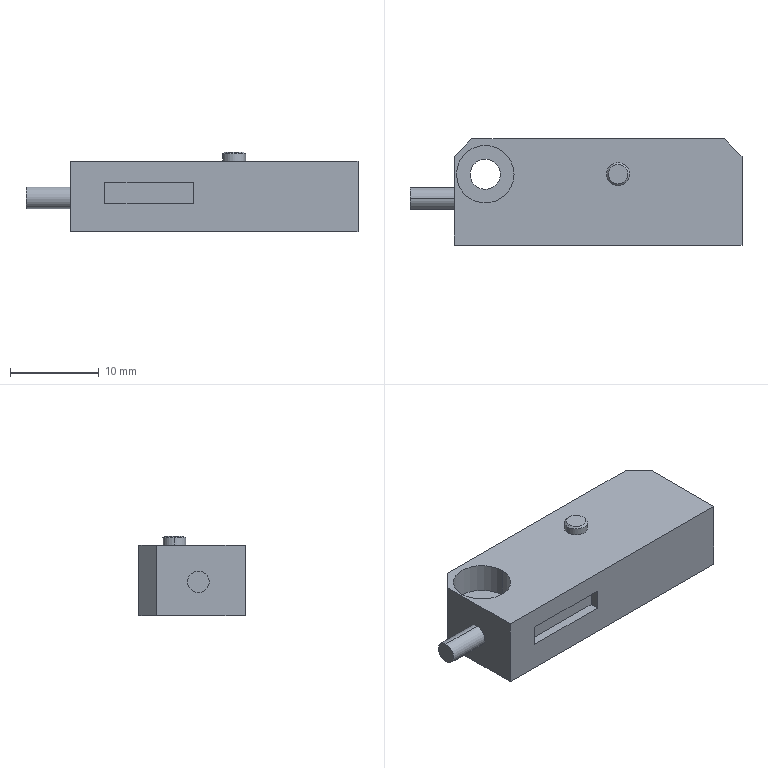Component | SolidWorks | FPJ-D21-1 | 1 solid | 26 faces | box 37.5 x 12 x 9 mm | volume 2938 mm3 | plane 16 | cylinder 8 | cone 2 | commonest cylinder face diameters 6.5 x2 3.4 x2 2.442 x2 2.6 x2
build123d program:
from build123d import *

# Parameters (mm, degrees)
SKETCH1_W                                       = 32.5
SKETCH1_H                                       = 12
BOSS_EXTRUDE1_DEPTH                             = 8
SKETCH2_R                                       = 1.3
BOSS_EXTRUDE2_DEPTH                             = 1
CHAMFER1_SIZE                                   = 2
SKETCH3_R                                       = 1.221
BOSS_EXTRUDE3_DEPTH                             = 5
M3_HEX_SOCKET_HEAD_CAP_SCREW_CBORE1_D           = 3.4
M3_HEX_SOCKET_HEAD_CAP_SCREW_CBORE1_CBORE_D     = 6.5
M3_HEX_SOCKET_HEAD_CAP_SCREW_CBORE1_CBORE_DEPTH = 3.4
BOSS_EXTRUDE4_START                             = 1
SKETCH6_R                                       = 1.3
BOSS_EXTRUDE4_DEPTH                             = 1
CHAMFER2_SIZE                                   = 0.2
SKETCH7_W                                       = 9.996
SKETCH7_H                                       = 2.373
CUT_EXTRUDE1_DEPTH                              = 1
PINSTUBRELIEF_SKETCH_R                          = 2
PINSTUBRELIEF_DEPTH                             = 2


with BuildPart() as part:
    # Sketch1 → Boss-Extrude1 (new body)
    with BuildSketch(Plane.XY):
        with Locations((-16.25, 6)):
            Rectangle(SKETCH1_W, SKETCH1_H)
    extrude(amount=BOSS_EXTRUDE1_DEPTH)

    # Sketch2 → Boss-Extrude2 (add)
    with BuildSketch(Plane.XY.offset(8)):
        with Locations((-14, 8)):
            Circle(SKETCH2_R)
    extrude(amount=BOSS_EXTRUDE2_DEPTH)

    # Chamfer1
    chamfer1_edges = [part.edges().sort_by_distance(p)[0] for p in [
        (-32.5, 12, 4),
        (0, 12, 4),
    ]]
    chamfer(chamfer1_edges, length=CHAMFER1_SIZE)

    # Sketch3 → Boss-Extrude3 (add)
    with BuildSketch(Plane.ZY.offset(32.5)):
        with Locations(Location((3.84, 5.275, 0), (0, 0, 180))):
            Circle(SKETCH3_R)
    extrude(amount=BOSS_EXTRUDE3_DEPTH)

    # M3 Hex Socket Head Cap Screw CBORE1 (through all)
    with Locations(Plane.XY.offset(8)):
        with Locations((-29, 8)):
            CounterBoreHole(M3_HEX_SOCKET_HEAD_CAP_SCREW_CBORE1_D / 2, M3_HEX_SOCKET_HEAD_CAP_SCREW_CBORE1_CBORE_D / 2, M3_HEX_SOCKET_HEAD_CAP_SCREW_CBORE1_CBORE_DEPTH)

    # Sketch6 → Boss-Extrude4 (add)
    with BuildSketch(Plane(origin=(0, 0, 0), x_dir=(-1, 0, 0), z_dir=(0, 0, -1)).offset(BOSS_EXTRUDE4_START)):
        with Locations(Location((14, 8, 0), (0, 0, 180))):
            Circle(SKETCH6_R)
    extrude(amount=-BOSS_EXTRUDE4_DEPTH)

    # Chamfer2
    chamfer2_edges = [part.edges().sort_by_distance(p)[0] for p in [
        (-15.3, 8, 9),
        (-15.3, 8, -1),
    ]]
    chamfer(chamfer2_edges, length=CHAMFER2_SIZE)

    # Sketch7 → Cut-Extrude1 (cut)
    with BuildSketch(Plane.XZ):
        with Locations((-23.593, 4.408)):
            Rectangle(SKETCH7_W, SKETCH7_H)
    extrude(amount=-CUT_EXTRUDE1_DEPTH, mode=Mode.SUBTRACT)

    # PinStubRelief_Sketch → PinStubRelief (cut)
    with BuildSketch(Plane.XY):
        with Locations((-14, 8)):
            Circle(PINSTUBRELIEF_SKETCH_R)
    extrude(amount=-PINSTUBRELIEF_DEPTH, mode=Mode.SUBTRACT)


solid = part.part

# Placed as in the assembly
solid = solid.moved(Location((215.5, -74, 1001.634), (0, 0, 0)))
STEP:
#1=COLOUR_RGB('',0.7922,0.8196,0.9333);
#2=FILL_AREA_STYLE_COLOUR('',#1);
#3=FILL_AREA_STYLE('',(#2));
#4=SURFACE_STYLE_FILL_AREA(#3);
#5=SURFACE_SIDE_STYLE('',(#4));
#6=SURFACE_STYLE_USAGE(.BOTH.,#5);
#7=PRESENTATION_STYLE_ASSIGNMENT((#6));
#8=CARTESIAN_POINT('',(7.976,-2.598,39.789));
#9=VERTEX_POINT('',#8);
#10=CARTESIAN_POINT('',(7.89,-2.598,39.789));
#11=VERTEX_POINT('',#10);
#12=CARTESIAN_POINT('',(7.933,-2.598,39.789));
#13=DIRECTION('',(0.,0.,1.));
#14=DIRECTION('',(1.,0.,0.));
#15=AXIS2_PLACEMENT_3D('',#12,#13,#14);
#16=CIRCLE('',#15,0.04331);
#17=EDGE_CURVE('',#9,#11,#16,.T.);
#18=ORIENTED_EDGE('',*,*,#17,.F.);
#19=CARTESIAN_POINT('',(7.984,-2.598,39.781));
#20=VERTEX_POINT('',#19);
#21=CARTESIAN_POINT('',(7.976,-2.598,39.789));
#22=DIRECTION('',(0.7071,0.,-0.7071));
#23=VECTOR('',#22,39.37);
#24=LINE('',#21,#23);
#25=EDGE_CURVE('',#9,#20,#24,.T.);
#26=ORIENTED_EDGE('',*,*,#25,.T.);
#27=CARTESIAN_POINT('',(7.882,-2.598,39.781));
#28=VERTEX_POINT('',#27);
#29=CARTESIAN_POINT('',(7.933,-2.598,39.781));
#30=DIRECTION('',(0.,0.,-1.));
#31=DIRECTION('',(1.,0.,0.));
#32=AXIS2_PLACEMENT_3D('',#29,#30,#31);
#33=CIRCLE('',#32,0.05118);
#34=EDGE_CURVE('',#28,#20,#33,.T.);
#35=ORIENTED_EDGE('',*,*,#34,.F.);
#36=CARTESIAN_POINT('',(7.89,-2.598,39.789));
#37=DIRECTION('',(-0.7071,0.,-0.7071));
#38=VECTOR('',#37,39.37);
#39=LINE('',#36,#38);
#40=EDGE_CURVE('',#11,#28,#39,.T.);
#41=ORIENTED_EDGE('',*,*,#40,.F.);
#42=EDGE_LOOP('',(#18,#26,#35,#41));
#43=FACE_OUTER_BOUND('',#42,.T.);
#44=CARTESIAN_POINT('',(7.933,-2.598,39.789));
#45=DIRECTION('',(0.,0.,-1.));
#46=DIRECTION('',(-1.,0.,0.));
#47=AXIS2_PLACEMENT_3D('',#44,#45,#46);
#48=CONICAL_SURFACE('',#47,0.04331,0.7854);
#49=ADVANCED_FACE('',(#43),#48,.T.);
#50=CARTESIAN_POINT('',(7.215,-2.598,39.616));
#51=VERTEX_POINT('',#50);
#52=CARTESIAN_POINT('',(7.47,-2.598,39.616));
#53=VERTEX_POINT('',#52);
#54=CARTESIAN_POINT('',(7.343,-2.598,39.616));
#55=DIRECTION('',(0.,0.,1.));
#56=DIRECTION('',(1.,0.,0.));
#57=AXIS2_PLACEMENT_3D('',#54,#55,#56);
#58=CIRCLE('',#57,0.128);
#59=EDGE_CURVE('',#51,#53,#58,.T.);
#60=ORIENTED_EDGE('',*,*,#59,.F.);
#61=CARTESIAN_POINT('',(7.215,-2.598,39.749));
#62=VERTEX_POINT('',#61);
#63=CARTESIAN_POINT('',(7.215,-2.598,39.749));
#64=DIRECTION('',(0.,0.,1.));
#65=VECTOR('',#64,39.37);
#66=LINE('',#63,#65);
#67=EDGE_CURVE('',#51,#62,#66,.T.);
#68=ORIENTED_EDGE('',*,*,#67,.T.);
#69=CARTESIAN_POINT('',(7.47,-2.598,39.749));
#70=VERTEX_POINT('',#69);
#71=CARTESIAN_POINT('',(7.343,-2.598,39.749));
#72=DIRECTION('',(0.,0.,1.));
#73=DIRECTION('',(1.,0.,0.));
#74=AXIS2_PLACEMENT_3D('',#71,#72,#73);
#75=CIRCLE('',#74,0.128);
#76=EDGE_CURVE('',#62,#70,#75,.T.);
#77=ORIENTED_EDGE('',*,*,#76,.T.);
#78=CARTESIAN_POINT('',(7.47,-2.598,39.749));
#79=DIRECTION('',(0.,0.,1.));
#80=VECTOR('',#79,39.37);
#81=LINE('',#78,#80);
#82=EDGE_CURVE('',#53,#70,#81,.T.);
#83=ORIENTED_EDGE('',*,*,#82,.F.);
#84=EDGE_LOOP('',(#60,#68,#77,#83));
#85=FACE_OUTER_BOUND('',#84,.T.);
#86=CARTESIAN_POINT('',(7.343,-2.598,39.749));
#87=DIRECTION('',(0.,0.,1.));
#88=DIRECTION('',(1.,0.,0.));
#89=AXIS2_PLACEMENT_3D('',#86,#87,#88);
#90=CYLINDRICAL_SURFACE('',#89,0.128);
#91=ADVANCED_FACE('',(#85),#90,.F.);
#92=CARTESIAN_POINT('',(7.276,-2.598,39.434));
#93=VERTEX_POINT('',#92);
#94=CARTESIAN_POINT('',(7.409,-2.598,39.434));
#95=VERTEX_POINT('',#94);
#96=CARTESIAN_POINT('',(7.343,-2.598,39.434));
#97=DIRECTION('',(0.,0.,1.));
#98=DIRECTION('',(1.,0.,0.));
#99=AXIS2_PLACEMENT_3D('',#96,#97,#98);
#100=CIRCLE('',#99,0.06693);
#101=EDGE_CURVE('',#93,#95,#100,.T.);
#102=ORIENTED_EDGE('',*,*,#101,.F.);
#103=CARTESIAN_POINT('',(7.276,-2.598,39.616));
#104=VERTEX_POINT('',#103);
#105=CARTESIAN_POINT('',(7.276,-2.598,39.749));
#106=DIRECTION('',(0.,0.,1.));
#107=VECTOR('',#106,39.37);
#108=LINE('',#105,#107);
#109=EDGE_CURVE('',#93,#104,#108,.T.);
#110=ORIENTED_EDGE('',*,*,#109,.T.);
#111=CARTESIAN_POINT('',(7.409,-2.598,39.616));
#112=VERTEX_POINT('',#111);
#113=CARTESIAN_POINT('',(7.343,-2.598,39.616));
#114=DIRECTION('',(0.,0.,1.));
#115=DIRECTION('',(1.,0.,0.));
#116=AXIS2_PLACEMENT_3D('',#113,#114,#115);
#117=CIRCLE('',#116,0.06693);
#118=EDGE_CURVE('',#104,#112,#117,.T.);
#119=ORIENTED_EDGE('',*,*,#118,.T.);
#120=CARTESIAN_POINT('',(7.409,-2.598,39.749));
#121=DIRECTION('',(0.,0.,1.));
#122=VECTOR('',#121,39.37);
#123=LINE('',#120,#122);
#124=EDGE_CURVE('',#95,#112,#123,.T.);
#125=ORIENTED_EDGE('',*,*,#124,.F.);
#126=EDGE_LOOP('',(#102,#110,#119,#125));
#127=FACE_OUTER_BOUND('',#126,.T.);
#128=CARTESIAN_POINT('',(7.343,-2.598,39.749));
#129=DIRECTION('',(0.,0.,1.));
#130=DIRECTION('',(1.,0.,0.));
#131=AXIS2_PLACEMENT_3D('',#128,#129,#130);
#132=CYLINDRICAL_SURFACE('',#131,0.06693);
#133=ADVANCED_FACE('',(#127),#132,.F.);
#134=CARTESIAN_POINT('',(7.008,-2.706,39.634));
#135=VERTEX_POINT('',#134);
#136=CARTESIAN_POINT('',(7.008,-2.706,39.538));
#137=VERTEX_POINT('',#136);
#138=CARTESIAN_POINT('',(7.008,-2.706,39.586));
#139=DIRECTION('',(-1.,0.,0.));
#140=DIRECTION('',(0.,0.,1.));
#141=AXIS2_PLACEMENT_3D('',#138,#139,#140);
#142=CIRCLE('',#141,0.04807);
#143=EDGE_CURVE('',#135,#137,#142,.T.);
#144=ORIENTED_EDGE('',*,*,#143,.F.);
#145=CARTESIAN_POINT('',(7.205,-2.706,39.634));
#146=VERTEX_POINT('',#145);
#147=CARTESIAN_POINT('',(7.008,-2.706,39.634));
#148=DIRECTION('',(1.,0.,0.));
#149=VECTOR('',#148,39.37);
#150=LINE('',#147,#149);
#151=EDGE_CURVE('',#135,#146,#150,.T.);
#152=ORIENTED_EDGE('',*,*,#151,.T.);
#153=CARTESIAN_POINT('',(7.205,-2.706,39.538));
#154=VERTEX_POINT('',#153);
#155=CARTESIAN_POINT('',(7.205,-2.706,39.586));
#156=DIRECTION('',(-1.,0.,0.));
#157=DIRECTION('',(0.,0.,-1.));
#158=AXIS2_PLACEMENT_3D('',#155,#156,#157);
#159=CIRCLE('',#158,0.04807);
#160=EDGE_CURVE('',#146,#154,#159,.T.);
#161=ORIENTED_EDGE('',*,*,#160,.T.);
#162=CARTESIAN_POINT('',(7.008,-2.706,39.538));
#163=DIRECTION('',(1.,0.,0.));
#164=VECTOR('',#163,39.37);
#165=LINE('',#162,#164);
#166=EDGE_CURVE('',#137,#154,#165,.T.);
#167=ORIENTED_EDGE('',*,*,#166,.F.);
#168=EDGE_LOOP('',(#144,#152,#161,#167));
#169=FACE_OUTER_BOUND('',#168,.T.);
#170=CARTESIAN_POINT('',(7.008,-2.706,39.586));
#171=DIRECTION('',(1.,0.,0.));
#172=DIRECTION('',(0.,0.,-1.));
#173=AXIS2_PLACEMENT_3D('',#170,#171,#172);
#174=CYLINDRICAL_SURFACE('',#173,0.04807);
#175=ADVANCED_FACE('',(#169),#174,.T.);
#176=ORIENTED_EDGE('',*,*,#34,.T.);
#177=CARTESIAN_POINT('',(7.984,-2.598,39.749));
#178=VERTEX_POINT('',#177);
#179=CARTESIAN_POINT('',(7.984,-2.598,39.789));
#180=DIRECTION('',(0.,0.,-1.));
#181=VECTOR('',#180,39.37);
#182=LINE('',#179,#181);
#183=EDGE_CURVE('',#20,#178,#182,.T.);
#184=ORIENTED_EDGE('',*,*,#183,.T.);
#185=CARTESIAN_POINT('',(7.882,-2.598,39.749));
#186=VERTEX_POINT('',#185);
#187=CARTESIAN_POINT('',(7.933,-2.598,39.749));
#188=DIRECTION('',(0.,0.,1.));
#189=DIRECTION('',(1.,0.,0.));
#190=AXIS2_PLACEMENT_3D('',#187,#188,#189);
#191=CIRCLE('',#190,0.05118);
#192=EDGE_CURVE('',#178,#186,#191,.T.);
#193=ORIENTED_EDGE('',*,*,#192,.T.);
#194=CARTESIAN_POINT('',(7.882,-2.598,39.789));
#195=DIRECTION('',(0.,0.,-1.));
#196=VECTOR('',#195,39.37);
#197=LINE('',#194,#196);
#198=EDGE_CURVE('',#28,#186,#197,.T.);
#199=ORIENTED_EDGE('',*,*,#198,.F.);
#200=EDGE_LOOP('',(#176,#184,#193,#199));
#201=FACE_OUTER_BOUND('',#200,.T.);
#202=CARTESIAN_POINT('',(7.933,-2.598,39.789));
#203=DIRECTION('',(0.,0.,-1.));
#204=DIRECTION('',(-1.,0.,0.));
#205=AXIS2_PLACEMENT_3D('',#202,#203,#204);
#206=CYLINDRICAL_SURFACE('',#205,0.05118);
#207=ADVANCED_FACE('',(#201),#206,.T.);
#208=CARTESIAN_POINT('',(7.343,-2.598,39.434));
#209=DIRECTION('',(0.,0.,1.));
#210=DIRECTION('',(1.,0.,0.));
#211=AXIS2_PLACEMENT_3D('',#208,#209,#210);
#212=CIRCLE('',#211,0.06693);
#213=EDGE_CURVE('',#95,#93,#212,.T.);
#214=ORIENTED_EDGE('',*,*,#213,.T.);
#215=ORIENTED_EDGE('',*,*,#101,.T.);
#216=EDGE_LOOP('',(#214,#215));
#217=FACE_BOUND('',#216,.T.);
#218=CARTESIAN_POINT('',(8.406,-2.441,39.434));
#219=VERTEX_POINT('',#218);
#220=CARTESIAN_POINT('',(7.283,-2.441,39.434));
#221=VERTEX_POINT('',#220);
#222=CARTESIAN_POINT('',(8.484,-2.441,39.434));
#223=DIRECTION('',(-1.,-0.,0.));
#224=VECTOR('',#223,39.37);
#225=LINE('',#222,#224);
#226=EDGE_CURVE('',#219,#221,#225,.T.);
#227=ORIENTED_EDGE('',*,*,#226,.F.);
#228=CARTESIAN_POINT('',(8.484,-2.52,39.434));
#229=VERTEX_POINT('',#228);
#230=CARTESIAN_POINT('',(8.406,-2.441,39.434));
#231=DIRECTION('',(0.7071,-0.7071,0.));
#232=VECTOR('',#231,39.37);
#233=LINE('',#230,#232);
#234=EDGE_CURVE('',#219,#229,#233,.T.);
#235=ORIENTED_EDGE('',*,*,#234,.T.);
#236=CARTESIAN_POINT('',(8.484,-2.913,39.434));
#237=VERTEX_POINT('',#236);
#238=CARTESIAN_POINT('',(8.484,-2.913,39.434));
#239=DIRECTION('',(0.,1.,0.));
#240=VECTOR('',#239,39.37);
#241=LINE('',#238,#240);
#242=EDGE_CURVE('',#237,#229,#241,.T.);
#243=ORIENTED_EDGE('',*,*,#242,.F.);
#244=CARTESIAN_POINT('',(7.205,-2.913,39.434));
#245=VERTEX_POINT('',#244);
#246=CARTESIAN_POINT('',(8.484,-2.913,39.434));
#247=DIRECTION('',(1.,0.,0.));
#248=VECTOR('',#247,39.37);
#249=LINE('',#246,#248);
#250=EDGE_CURVE('',#245,#237,#249,.T.);
#251=ORIENTED_EDGE('',*,*,#250,.F.);
#252=CARTESIAN_POINT('',(7.205,-2.52,39.434));
#253=VERTEX_POINT('',#252);
#254=CARTESIAN_POINT('',(7.205,-2.913,39.434));
#255=DIRECTION('',(0.,-1.,0.));
#256=VECTOR('',#255,39.37);
#257=LINE('',#254,#256);
#258=EDGE_CURVE('',#253,#245,#257,.T.);
#259=ORIENTED_EDGE('',*,*,#258,.F.);
#260=CARTESIAN_POINT('',(7.205,-2.52,39.434));
#261=DIRECTION('',(0.7071,0.7071,0.));
#262=VECTOR('',#261,39.37);
#263=LINE('',#260,#262);
#264=EDGE_CURVE('',#253,#221,#263,.T.);
#265=ORIENTED_EDGE('',*,*,#264,.T.);
#266=EDGE_LOOP('',(#227,#235,#243,#251,#259,#265));
#267=FACE_OUTER_BOUND('',#266,.T.);
#268=CARTESIAN_POINT('',(8.484,-2.913,39.434));
#269=DIRECTION('',(0.,0.,1.));
#270=DIRECTION('',(1.,0.,0.));
#271=AXIS2_PLACEMENT_3D('',#268,#269,#270);
#272=PLANE('',#271);
#273=ADVANCED_FACE('',(#217,#267),#272,.F.);
#274=CARTESIAN_POINT('',(7.205,-2.52,39.749));
#275=VERTEX_POINT('',#274);
#276=CARTESIAN_POINT('',(7.205,-2.913,39.749));
#277=VERTEX_POINT('',#276);
#278=CARTESIAN_POINT('',(7.205,-2.913,39.749));
#279=DIRECTION('',(0.,-1.,0.));
#280=VECTOR('',#279,39.37);
#281=LINE('',#278,#280);
#282=EDGE_CURVE('',#275,#277,#281,.T.);
#283=ORIENTED_EDGE('',*,*,#282,.F.);
#284=CARTESIAN_POINT('',(7.205,-2.52,39.749));
#285=DIRECTION('',(0.,0.,-1.));
#286=VECTOR('',#285,39.37);
#287=LINE('',#284,#286);
#288=EDGE_CURVE('',#275,#253,#287,.T.);
#289=ORIENTED_EDGE('',*,*,#288,.T.);
#290=ORIENTED_EDGE('',*,*,#258,.T.);
#291=CARTESIAN_POINT('',(7.205,-2.913,39.749));
#292=DIRECTION('',(0.,0.,-1.));
#293=VECTOR('',#292,39.37);
#294=LINE('',#291,#293);
#295=EDGE_CURVE('',#277,#245,#294,.T.);
#296=ORIENTED_EDGE('',*,*,#295,.F.);
#297=EDGE_LOOP('',(#283,#289,#290,#296));
#298=FACE_OUTER_BOUND('',#297,.T.);
#299=CARTESIAN_POINT('',(7.205,-2.706,39.586));
#300=DIRECTION('',(-1.,0.,0.));
#301=DIRECTION('',(0.,0.,-1.));
#302=AXIS2_PLACEMENT_3D('',#299,#300,#301);
#303=CIRCLE('',#302,0.04807);
#304=EDGE_CURVE('',#154,#146,#303,.T.);
#305=ORIENTED_EDGE('',*,*,#304,.F.);
#306=ORIENTED_EDGE('',*,*,#160,.F.);
#307=EDGE_LOOP('',(#305,#306));
#308=FACE_BOUND('',#307,.T.);
#309=CARTESIAN_POINT('',(7.205,-2.913,39.749));
#310=DIRECTION('',(1.,0.,0.));
#311=DIRECTION('',(0.,0.,-1.));
#312=AXIS2_PLACEMENT_3D('',#309,#310,#311);
#313=PLANE('',#312);
#314=ADVANCED_FACE('',(#298,#308),#313,.F.);
#315=CARTESIAN_POINT('',(7.343,-2.598,39.749));
#316=DIRECTION('',(0.,0.,1.));
#317=DIRECTION('',(1.,0.,0.));
#318=AXIS2_PLACEMENT_3D('',#315,#316,#317);
#319=CIRCLE('',#318,0.128);
#320=EDGE_CURVE('',#70,#62,#319,.T.);
#321=ORIENTED_EDGE('',*,*,#320,.F.);
#322=ORIENTED_EDGE('',*,*,#76,.F.);
#323=EDGE_LOOP('',(#321,#322));
#324=FACE_BOUND('',#323,.T.);
#325=CARTESIAN_POINT('',(8.484,-2.913,39.749));
#326=VERTEX_POINT('',#325);
#327=CARTESIAN_POINT('',(8.484,-2.52,39.749));
#328=VERTEX_POINT('',#327);
#329=CARTESIAN_POINT('',(8.484,-2.913,39.749));
#330=DIRECTION('',(0.,1.,0.));
#331=VECTOR('',#330,39.37);
#332=LINE('',#329,#331);
#333=EDGE_CURVE('',#326,#328,#332,.T.);
#334=ORIENTED_EDGE('',*,*,#333,.T.);
#335=CARTESIAN_POINT('',(8.406,-2.441,39.749));
#336=VERTEX_POINT('',#335);
#337=CARTESIAN_POINT('',(8.681,-2.717,39.749));
#338=DIRECTION('',(-0.7071,0.7071,0.));
#339=VECTOR('',#338,39.37);
#340=LINE('',#337,#339);
#341=EDGE_CURVE('',#328,#336,#340,.T.);
#342=ORIENTED_EDGE('',*,*,#341,.T.);
#343=CARTESIAN_POINT('',(7.283,-2.441,39.749));
#344=VERTEX_POINT('',#343);
#345=CARTESIAN_POINT('',(8.484,-2.441,39.749));
#346=DIRECTION('',(-1.,-0.,0.));
#347=VECTOR('',#346,39.37);
#348=LINE('',#345,#347);
#349=EDGE_CURVE('',#336,#344,#348,.T.);
#350=ORIENTED_EDGE('',*,*,#349,.T.);
#351=CARTESIAN_POINT('',(7.648,-2.077,39.749));
#352=DIRECTION('',(-0.7071,-0.7071,0.));
#353=VECTOR('',#352,39.37);
#354=LINE('',#351,#353);
#355=EDGE_CURVE('',#344,#275,#354,.T.);
#356=ORIENTED_EDGE('',*,*,#355,.T.);
#357=ORIENTED_EDGE('',*,*,#282,.T.);
#358=CARTESIAN_POINT('',(8.484,-2.913,39.749));
#359=DIRECTION('',(1.,0.,0.));
#360=VECTOR('',#359,39.37);
#361=LINE('',#358,#360);
#362=EDGE_CURVE('',#277,#326,#361,.T.);
#363=ORIENTED_EDGE('',*,*,#362,.T.);
#364=EDGE_LOOP('',(#334,#342,#350,#356,#357,#363));
#365=FACE_OUTER_BOUND('',#364,.T.);
#366=CARTESIAN_POINT('',(7.933,-2.598,39.749));
#367=DIRECTION('',(0.,0.,1.));
#368=DIRECTION('',(1.,0.,0.));
#369=AXIS2_PLACEMENT_3D('',#366,#367,#368);
#370=CIRCLE('',#369,0.05118);
#371=EDGE_CURVE('',#186,#178,#370,.T.);
#372=ORIENTED_EDGE('',*,*,#371,.F.);
#373=ORIENTED_EDGE('',*,*,#192,.F.);
#374=EDGE_LOOP('',(#372,#373));
#375=FACE_BOUND('',#374,.T.);
#376=CARTESIAN_POINT('',(8.484,-2.913,39.749));
#377=DIRECTION('',(0.,0.,1.));
#378=DIRECTION('',(1.,0.,0.));
#379=AXIS2_PLACEMENT_3D('',#376,#377,#378);
#380=PLANE('',#379);
#381=ADVANCED_FACE('',(#324,#365,#375),#380,.T.);
#382=ORIENTED_EDGE('',*,*,#242,.T.);
#383=CARTESIAN_POINT('',(8.484,-2.52,39.749));
#384=DIRECTION('',(0.,0.,1.));
#385=VECTOR('',#384,39.37);
#386=LINE('',#383,#385);
#387=EDGE_CURVE('',#229,#328,#386,.T.);
#388=ORIENTED_EDGE('',*,*,#387,.T.);
#389=ORIENTED_EDGE('',*,*,#333,.F.);
#390=CARTESIAN_POINT('',(8.484,-2.913,39.749));
#391=DIRECTION('',(0.,0.,-1.));
#392=VECTOR('',#391,39.37);
#393=LINE('',#390,#392);
#394=EDGE_CURVE('',#326,#237,#393,.T.);
#395=ORIENTED_EDGE('',*,*,#394,.T.);
#396=EDGE_LOOP('',(#382,#388,#389,#395));
#397=FACE_OUTER_BOUND('',#396,.T.);
#398=CARTESIAN_POINT('',(8.484,-2.913,39.749));
#399=DIRECTION('',(-1.,0.,0.));
#400=DIRECTION('',(0.,0.,1.));
#401=AXIS2_PLACEMENT_3D('',#398,#399,#400);
#402=PLANE('',#401);
#403=ADVANCED_FACE('',(#397),#402,.F.);
#404=ORIENTED_EDGE('',*,*,#349,.F.);
#405=CARTESIAN_POINT('',(8.406,-2.441,39.749));
#406=DIRECTION('',(0.,0.,-1.));
#407=VECTOR('',#406,39.37);
#408=LINE('',#405,#407);
#409=EDGE_CURVE('',#336,#219,#408,.T.);
#410=ORIENTED_EDGE('',*,*,#409,.T.);
#411=ORIENTED_EDGE('',*,*,#226,.T.);
#412=CARTESIAN_POINT('',(7.283,-2.441,39.749));
#413=DIRECTION('',(0.,0.,1.));
#414=VECTOR('',#413,39.37);
#415=LINE('',#412,#414);
#416=EDGE_CURVE('',#221,#344,#415,.T.);
#417=ORIENTED_EDGE('',*,*,#416,.T.);
#418=EDGE_LOOP('',(#404,#410,#411,#417));
#419=FACE_OUTER_BOUND('',#418,.T.);
#420=CARTESIAN_POINT('',(8.484,-2.441,39.749));
#421=DIRECTION('',(0.,-1.,0.));
#422=DIRECTION('',(1.,0.,0.));
#423=AXIS2_PLACEMENT_3D('',#420,#421,#422);
#424=PLANE('',#423);
#425=ADVANCED_FACE('',(#419),#424,.F.);
#426=CARTESIAN_POINT('',(7.359,-2.913,39.561));
#427=VERTEX_POINT('',#426);
#428=CARTESIAN_POINT('',(7.752,-2.913,39.561));
#429=VERTEX_POINT('',#428);
#430=CARTESIAN_POINT('',(7.359,-2.913,39.561));
#431=DIRECTION('',(1.,0.,0.));
#432=VECTOR('',#431,39.37);
#433=LINE('',#430,#432);
#434=EDGE_CURVE('',#427,#429,#433,.T.);
#435=ORIENTED_EDGE('',*,*,#434,.F.);
#436=CARTESIAN_POINT('',(7.359,-2.913,39.655));
#437=VERTEX_POINT('',#436);
#438=CARTESIAN_POINT('',(7.359,-2.913,39.655));
#439=DIRECTION('',(0.,0.,-1.));
#440=VECTOR('',#439,39.37);
#441=LINE('',#438,#440);
#442=EDGE_CURVE('',#437,#427,#441,.T.);
#443=ORIENTED_EDGE('',*,*,#442,.F.);
#444=CARTESIAN_POINT('',(7.752,-2.913,39.655));
#445=VERTEX_POINT('',#444);
#446=CARTESIAN_POINT('',(7.359,-2.913,39.655));
#447=DIRECTION('',(-1.,-0.,0.));
#448=VECTOR('',#447,39.37);
#449=LINE('',#446,#448);
#450=EDGE_CURVE('',#445,#437,#449,.T.);
#451=ORIENTED_EDGE('',*,*,#450,.F.);
#452=CARTESIAN_POINT('',(7.752,-2.913,39.655));
#453=DIRECTION('',(0.,0.,1.));
#454=VECTOR('',#453,39.37);
#455=LINE('',#452,#454);
#456=EDGE_CURVE('',#429,#445,#455,.T.);
#457=ORIENTED_EDGE('',*,*,#456,.F.);
#458=EDGE_LOOP('',(#435,#443,#451,#457));
#459=FACE_BOUND('',#458,.T.);
#460=ORIENTED_EDGE('',*,*,#250,.T.);
#461=ORIENTED_EDGE('',*,*,#394,.F.);
#462=ORIENTED_EDGE('',*,*,#362,.F.);
#463=ORIENTED_EDGE('',*,*,#295,.T.);
#464=EDGE_LOOP('',(#460,#461,#462,#463));
#465=FACE_OUTER_BOUND('',#464,.T.);
#466=CARTESIAN_POINT('',(8.484,-2.913,39.749));
#467=DIRECTION('',(-0.,1.,0.));
#468=DIRECTION('',(-1.,-0.,0.));
#469=AXIS2_PLACEMENT_3D('',#466,#467,#468);
#470=PLANE('',#469);
#471=ADVANCED_FACE('',(#459,#465),#470,.F.);
#472=ORIENTED_EDGE('',*,*,#183,.F.);
#473=CARTESIAN_POINT('',(7.933,-2.598,39.781));
#474=DIRECTION('',(0.,0.,-1.));
#475=DIRECTION('',(1.,0.,0.));
#476=AXIS2_PLACEMENT_3D('',#473,#474,#475);
#477=CIRCLE('',#476,0.05118);
#478=EDGE_CURVE('',#20,#28,#477,.T.);
#479=ORIENTED_EDGE('',*,*,#478,.T.);
#480=ORIENTED_EDGE('',*,*,#198,.T.);
#481=ORIENTED_EDGE('',*,*,#371,.T.);
#482=EDGE_LOOP('',(#472,#479,#480,#481));
#483=FACE_OUTER_BOUND('',#482,.T.);
#484=CARTESIAN_POINT('',(7.933,-2.598,39.789));
#485=DIRECTION('',(0.,0.,-1.));
#486=DIRECTION('',(-1.,0.,0.));
#487=AXIS2_PLACEMENT_3D('',#484,#485,#486);
#488=CYLINDRICAL_SURFACE('',#487,0.05118);
#489=ADVANCED_FACE('',(#483),#488,.T.);
#490=CARTESIAN_POINT('',(7.933,-2.598,39.789));
#491=DIRECTION('',(0.,0.,1.));
#492=DIRECTION('',(1.,0.,0.));
#493=AXIS2_PLACEMENT_3D('',#490,#491,#492);
#494=CIRCLE('',#493,0.04331);
#495=EDGE_CURVE('',#11,#9,#494,.T.);
#496=ORIENTED_EDGE('',*,*,#495,.T.);
#497=ORIENTED_EDGE('',*,*,#17,.T.);
#498=EDGE_LOOP('',(#496,#497));
#499=FACE_OUTER_BOUND('',#498,.T.);
#500=CARTESIAN_POINT('',(7.933,-2.598,39.789));
#501=DIRECTION('',(0.,0.,1.));
#502=DIRECTION('',(1.,0.,0.));
#503=AXIS2_PLACEMENT_3D('',#500,#501,#502);
#504=PLANE('',#503);
#505=ADVANCED_FACE('',(#499),#504,.T.);
#506=ORIENTED_EDGE('',*,*,#341,.F.);
#507=ORIENTED_EDGE('',*,*,#387,.F.);
#508=ORIENTED_EDGE('',*,*,#234,.F.);
#509=ORIENTED_EDGE('',*,*,#409,.F.);
#510=EDGE_LOOP('',(#506,#507,#508,#509));
#511=FACE_OUTER_BOUND('',#510,.T.);
#512=CARTESIAN_POINT('',(8.406,-2.441,39.749));
#513=DIRECTION('',(-0.7071,-0.7071,0.));
#514=DIRECTION('',(0.,0.,-1.));
#515=AXIS2_PLACEMENT_3D('',#512,#513,#514);
#516=PLANE('',#515);
#517=ADVANCED_FACE('',(#511),#516,.F.);
#518=ORIENTED_EDGE('',*,*,#355,.F.);
#519=ORIENTED_EDGE('',*,*,#416,.F.);
#520=ORIENTED_EDGE('',*,*,#264,.F.);
#521=ORIENTED_EDGE('',*,*,#288,.F.);
#522=EDGE_LOOP('',(#518,#519,#520,#521));
#523=FACE_OUTER_BOUND('',#522,.T.);
#524=CARTESIAN_POINT('',(7.205,-2.52,39.749));
#525=DIRECTION('',(0.7071,-0.7071,0.));
#526=DIRECTION('',(0.,0.,-1.));
#527=AXIS2_PLACEMENT_3D('',#524,#525,#526);
#528=PLANE('',#527);
#529=ADVANCED_FACE('',(#523),#528,.F.);
#530=ORIENTED_EDGE('',*,*,#151,.F.);
#531=CARTESIAN_POINT('',(7.008,-2.706,39.586));
#532=DIRECTION('',(-1.,0.,0.));
#533=DIRECTION('',(0.,0.,1.));
#534=AXIS2_PLACEMENT_3D('',#531,#532,#533);
#535=CIRCLE('',#534,0.04807);
#536=EDGE_CURVE('',#137,#135,#535,.T.);
#537=ORIENTED_EDGE('',*,*,#536,.F.);
#538=ORIENTED_EDGE('',*,*,#166,.T.);
#539=ORIENTED_EDGE('',*,*,#304,.T.);
#540=EDGE_LOOP('',(#530,#537,#538,#539));
#541=FACE_OUTER_BOUND('',#540,.T.);
#542=CARTESIAN_POINT('',(7.008,-2.706,39.586));
#543=DIRECTION('',(1.,0.,0.));
#544=DIRECTION('',(0.,0.,-1.));
#545=AXIS2_PLACEMENT_3D('',#542,#543,#544);
#546=CYLINDRICAL_SURFACE('',#545,0.04807);
#547=ADVANCED_FACE('',(#541),#546,.T.);
#548=ORIENTED_EDGE('',*,*,#536,.T.);
#549=ORIENTED_EDGE('',*,*,#143,.T.);
#550=EDGE_LOOP('',(#548,#549));
#551=FACE_OUTER_BOUND('',#550,.T.);
#552=CARTESIAN_POINT('',(7.008,-2.706,39.586));
#553=DIRECTION('',(-1.,0.,0.));
#554=DIRECTION('',(0.,0.,1.));
#555=AXIS2_PLACEMENT_3D('',#552,#553,#554);
#556=PLANE('',#555);
#557=ADVANCED_FACE('',(#551),#556,.T.);
#558=ORIENTED_EDGE('',*,*,#109,.F.);
#559=ORIENTED_EDGE('',*,*,#213,.F.);
#560=ORIENTED_EDGE('',*,*,#124,.T.);
#561=CARTESIAN_POINT('',(7.343,-2.598,39.616));
#562=DIRECTION('',(0.,0.,1.));
#563=DIRECTION('',(1.,0.,0.));
#564=AXIS2_PLACEMENT_3D('',#561,#562,#563);
#565=CIRCLE('',#564,0.06693);
#566=EDGE_CURVE('',#112,#104,#565,.T.);
#567=ORIENTED_EDGE('',*,*,#566,.T.);
#568=EDGE_LOOP('',(#558,#559,#560,#567));
#569=FACE_OUTER_BOUND('',#568,.T.);
#570=CARTESIAN_POINT('',(7.343,-2.598,39.749));
#571=DIRECTION('',(0.,0.,1.));
#572=DIRECTION('',(1.,0.,0.));
#573=AXIS2_PLACEMENT_3D('',#570,#571,#572);
#574=CYLINDRICAL_SURFACE('',#573,0.06693);
#575=ADVANCED_FACE('',(#569),#574,.F.);
#576=ORIENTED_EDGE('',*,*,#566,.F.);
#577=ORIENTED_EDGE('',*,*,#118,.F.);
#578=EDGE_LOOP('',(#576,#577));
#579=FACE_BOUND('',#578,.T.);
#580=CARTESIAN_POINT('',(7.343,-2.598,39.616));
#581=DIRECTION('',(0.,0.,1.));
#582=DIRECTION('',(1.,0.,0.));
#583=AXIS2_PLACEMENT_3D('',#580,#581,#582);
#584=CIRCLE('',#583,0.128);
#585=EDGE_CURVE('',#53,#51,#584,.T.);
#586=ORIENTED_EDGE('',*,*,#585,.T.);
#587=ORIENTED_EDGE('',*,*,#59,.T.);
#588=EDGE_LOOP('',(#586,#587));
#589=FACE_OUTER_BOUND('',#588,.T.);
#590=CARTESIAN_POINT('',(7.409,-2.598,39.616));
#591=DIRECTION('',(0.,0.,-1.));
#592=DIRECTION('',(-1.,0.,0.));
#593=AXIS2_PLACEMENT_3D('',#590,#591,#592);
#594=PLANE('',#593);
#595=ADVANCED_FACE('',(#579,#589),#594,.F.);
#596=ORIENTED_EDGE('',*,*,#67,.F.);
#597=ORIENTED_EDGE('',*,*,#585,.F.);
#598=ORIENTED_EDGE('',*,*,#82,.T.);
#599=ORIENTED_EDGE('',*,*,#320,.T.);
#600=EDGE_LOOP('',(#596,#597,#598,#599));
#601=FACE_OUTER_BOUND('',#600,.T.);
#602=CARTESIAN_POINT('',(7.343,-2.598,39.749));
#603=DIRECTION('',(0.,0.,1.));
#604=DIRECTION('',(1.,0.,0.));
#605=AXIS2_PLACEMENT_3D('',#602,#603,#604);
#606=CYLINDRICAL_SURFACE('',#605,0.128);
#607=ADVANCED_FACE('',(#601),#606,.F.);
#608=ORIENTED_EDGE('',*,*,#25,.F.);
#609=ORIENTED_EDGE('',*,*,#495,.F.);
#610=ORIENTED_EDGE('',*,*,#40,.T.);
#611=ORIENTED_EDGE('',*,*,#478,.F.);
#612=EDGE_LOOP('',(#608,#609,#610,#611));
#613=FACE_OUTER_BOUND('',#612,.T.);
#614=CARTESIAN_POINT('',(7.933,-2.598,39.789));
#615=DIRECTION('',(0.,0.,-1.));
#616=DIRECTION('',(-1.,0.,0.));
#617=AXIS2_PLACEMENT_3D('',#614,#615,#616);
#618=CONICAL_SURFACE('',#617,0.04331,0.7854);
#619=ADVANCED_FACE('',(#613),#618,.T.);
#620=ORIENTED_EDGE('',*,*,#442,.T.);
#621=CARTESIAN_POINT('',(7.359,-2.874,39.561));
#622=VERTEX_POINT('',#621);
#623=CARTESIAN_POINT('',(7.359,-2.874,39.561));
#624=DIRECTION('',(0.,-1.,0.));
#625=VECTOR('',#624,39.37);
#626=LINE('',#623,#625);
#627=EDGE_CURVE('',#622,#427,#626,.T.);
#628=ORIENTED_EDGE('',*,*,#627,.F.);
#629=CARTESIAN_POINT('',(7.359,-2.874,39.655));
#630=VERTEX_POINT('',#629);
#631=CARTESIAN_POINT('',(7.359,-2.874,39.655));
#632=DIRECTION('',(0.,0.,-1.));
#633=VECTOR('',#632,39.37);
#634=LINE('',#631,#633);
#635=EDGE_CURVE('',#630,#622,#634,.T.);
#636=ORIENTED_EDGE('',*,*,#635,.F.);
#637=CARTESIAN_POINT('',(7.359,-2.874,39.655));
#638=DIRECTION('',(0.,-1.,0.));
#639=VECTOR('',#638,39.37);
#640=LINE('',#637,#639);
#641=EDGE_CURVE('',#630,#437,#640,.T.);
#642=ORIENTED_EDGE('',*,*,#641,.T.);
#643=EDGE_LOOP('',(#620,#628,#636,#642));
#644=FACE_OUTER_BOUND('',#643,.T.);
#645=CARTESIAN_POINT('',(7.359,-2.874,39.655));
#646=DIRECTION('',(-1.,-0.,0.));
#647=DIRECTION('',(0.,-1.,0.));
#648=AXIS2_PLACEMENT_3D('',#645,#646,#647);
#649=PLANE('',#648);
#650=ADVANCED_FACE('',(#644),#649,.F.);
#651=ORIENTED_EDGE('',*,*,#450,.T.);
#652=ORIENTED_EDGE('',*,*,#641,.F.);
#653=CARTESIAN_POINT('',(7.752,-2.874,39.655));
#654=VERTEX_POINT('',#653);
#655=CARTESIAN_POINT('',(7.359,-2.874,39.655));
#656=DIRECTION('',(-1.,-0.,0.));
#657=VECTOR('',#656,39.37);
#658=LINE('',#655,#657);
#659=EDGE_CURVE('',#654,#630,#658,.T.);
#660=ORIENTED_EDGE('',*,*,#659,.F.);
#661=CARTESIAN_POINT('',(7.752,-2.874,39.655));
#662=DIRECTION('',(0.,-1.,0.));
#663=VECTOR('',#662,39.37);
#664=LINE('',#661,#663);
#665=EDGE_CURVE('',#654,#445,#664,.T.);
#666=ORIENTED_EDGE('',*,*,#665,.T.);
#667=EDGE_LOOP('',(#651,#652,#660,#666));
#668=FACE_OUTER_BOUND('',#667,.T.);
#669=CARTESIAN_POINT('',(7.359,-2.874,39.655));
#670=DIRECTION('',(0.,0.,1.));
#671=DIRECTION('',(1.,0.,0.));
#672=AXIS2_PLACEMENT_3D('',#669,#670,#671);
#673=PLANE('',#672);
#674=ADVANCED_FACE('',(#668),#673,.F.);
#675=ORIENTED_EDGE('',*,*,#456,.T.);
#676=ORIENTED_EDGE('',*,*,#665,.F.);
#677=CARTESIAN_POINT('',(7.752,-2.874,39.561));
#678=VERTEX_POINT('',#677);
#679=CARTESIAN_POINT('',(7.752,-2.874,39.655));
#680=DIRECTION('',(0.,0.,1.));
#681=VECTOR('',#680,39.37);
#682=LINE('',#679,#681);
#683=EDGE_CURVE('',#678,#654,#682,.T.);
#684=ORIENTED_EDGE('',*,*,#683,.F.);
#685=CARTESIAN_POINT('',(7.752,-2.874,39.561));
#686=DIRECTION('',(0.,-1.,0.));
#687=VECTOR('',#686,39.37);
#688=LINE('',#685,#687);
#689=EDGE_CURVE('',#678,#429,#688,.T.);
#690=ORIENTED_EDGE('',*,*,#689,.T.);
#691=EDGE_LOOP('',(#675,#676,#684,#690));
#692=FACE_OUTER_BOUND('',#691,.T.);
#693=CARTESIAN_POINT('',(7.752,-2.874,39.655));
#694=DIRECTION('',(1.,0.,0.));
#695=DIRECTION('',(-0.,1.,0.));
#696=AXIS2_PLACEMENT_3D('',#693,#694,#695);
#697=PLANE('',#696);
#698=ADVANCED_FACE('',(#692),#697,.F.);
#699=ORIENTED_EDGE('',*,*,#434,.T.);
#700=ORIENTED_EDGE('',*,*,#689,.F.);
#701=CARTESIAN_POINT('',(7.359,-2.874,39.561));
#702=DIRECTION('',(1.,0.,0.));
#703=VECTOR('',#702,39.37);
#704=LINE('',#701,#703);
#705=EDGE_CURVE('',#622,#678,#704,.T.);
#706=ORIENTED_EDGE('',*,*,#705,.F.);
#707=ORIENTED_EDGE('',*,*,#627,.T.);
#708=EDGE_LOOP('',(#699,#700,#706,#707));
#709=FACE_OUTER_BOUND('',#708,.T.);
#710=CARTESIAN_POINT('',(7.359,-2.874,39.561));
#711=DIRECTION('',(0.,0.,-1.));
#712=DIRECTION('',(-1.,0.,0.));
#713=AXIS2_PLACEMENT_3D('',#710,#711,#712);
#714=PLANE('',#713);
#715=ADVANCED_FACE('',(#709),#714,.F.);
#716=ORIENTED_EDGE('',*,*,#635,.T.);
#717=ORIENTED_EDGE('',*,*,#705,.T.);
#718=ORIENTED_EDGE('',*,*,#683,.T.);
#719=ORIENTED_EDGE('',*,*,#659,.T.);
#720=EDGE_LOOP('',(#716,#717,#718,#719));
#721=FACE_OUTER_BOUND('',#720,.T.);
#722=CARTESIAN_POINT('',(8.484,-2.874,39.434));
#723=DIRECTION('',(0.,-1.,0.));
#724=DIRECTION('',(1.,0.,0.));
#725=AXIS2_PLACEMENT_3D('',#722,#723,#724);
#726=PLANE('',#725);
#727=ADVANCED_FACE('',(#721),#726,.T.);
#728=CLOSED_SHELL('',(#49,#91,#133,#175,#207,#273,#314,#381,#403,#425,#471,#489,#505,#517,#529,#547,#557,#575,#595,#607,#619,#650,#674,#698,#715,#727));
#729=MANIFOLD_SOLID_BREP('',#728);
#730=STYLED_ITEM('',(#7),#729);
#731=PRESENTATION_LAYER_ASSIGNMENT('','',(#730));
#732=CARTESIAN_POINT('',(0.,0.,0.));
#733=DIRECTION('',(0.,0.,1.));
#734=DIRECTION('',(1.,0.,0.));
#735=AXIS2_PLACEMENT_3D('',#732,#733,#734);
#736=(LENGTH_UNIT()NAMED_UNIT(*)SI_UNIT($,.METRE.));
#737=LENGTH_MEASURE_WITH_UNIT(LENGTH_MEASURE(0.0254),#736);
#738=DIMENSIONAL_EXPONENTS(1.,0.,0.,0.,0.,0.,0.);
#739=(CONVERSION_BASED_UNIT('',#737)LENGTH_UNIT()NAMED_UNIT(#738));
#740=UNCERTAINTY_MEASURE_WITH_UNIT(LENGTH_MEASURE(0.00001),#739,'','');
#741=(NAMED_UNIT(*)PLANE_ANGLE_UNIT()SI_UNIT($,.RADIAN.));
#742=(NAMED_UNIT(*)SI_UNIT($,.STERADIAN.)SOLID_ANGLE_UNIT());
#743=(GEOMETRIC_REPRESENTATION_CONTEXT(3)GLOBAL_UNCERTAINTY_ASSIGNED_CONTEXT((#740))GLOBAL_UNIT_ASSIGNED_CONTEXT((#739,#741,#742))REPRESENTATION_CONTEXT('',''));
#744=ADVANCED_BREP_SHAPE_REPRESENTATION('',(#729,#735),#743);
#745=(LENGTH_UNIT()NAMED_UNIT(*)SI_UNIT($,.METRE.));
#746=LENGTH_MEASURE_WITH_UNIT(LENGTH_MEASURE(0.0254),#745);
#747=DIMENSIONAL_EXPONENTS(1.,0.,0.,0.,0.,0.,0.);
#748=(CONVERSION_BASED_UNIT('',#746)LENGTH_UNIT()NAMED_UNIT(#747));
#749=UNCERTAINTY_MEASURE_WITH_UNIT(LENGTH_MEASURE(0.00001),#748,'','');
#750=(NAMED_UNIT(*)PLANE_ANGLE_UNIT()SI_UNIT($,.RADIAN.));
#751=(NAMED_UNIT(*)SI_UNIT($,.STERADIAN.)SOLID_ANGLE_UNIT());
#752=(GEOMETRIC_REPRESENTATION_CONTEXT(3)GLOBAL_UNCERTAINTY_ASSIGNED_CONTEXT((#749))GLOBAL_UNIT_ASSIGNED_CONTEXT((#748,#750,#751))REPRESENTATION_CONTEXT('',''));
#753=MECHANICAL_DESIGN_GEOMETRIC_PRESENTATION_REPRESENTATION('',(#730),#752);